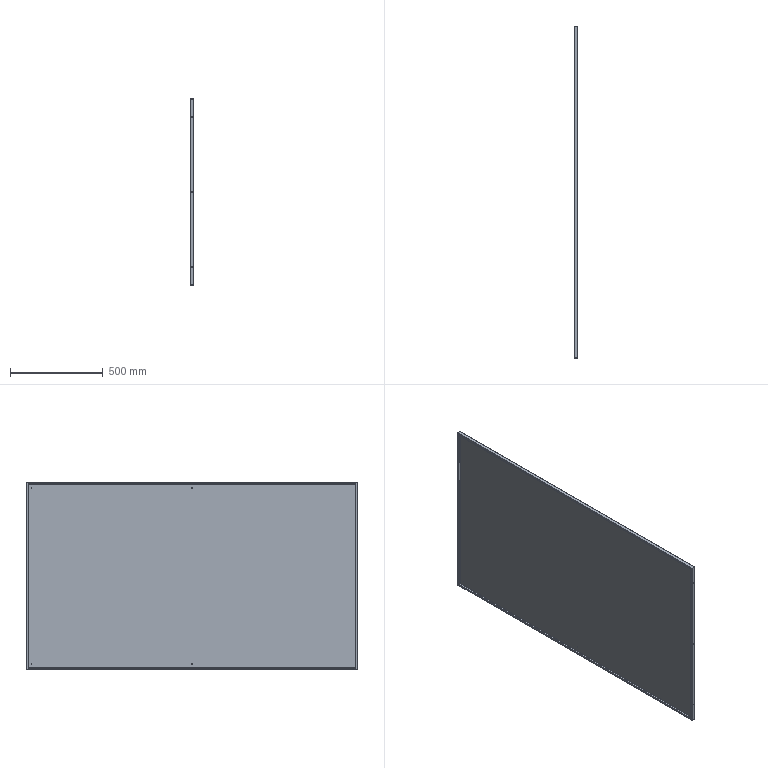Component | SolidWorks | RearDoorPanelWeldment-1_RearDoorPanel-1 | 1 solid | 112 faces | volume 2150851 mm3 | cylinder 54 | plane 46 | spline 12 | commonest cylinder face diameters 3 x24 2.5 x8 0.2 x8 2.4 x8 5.2 x6